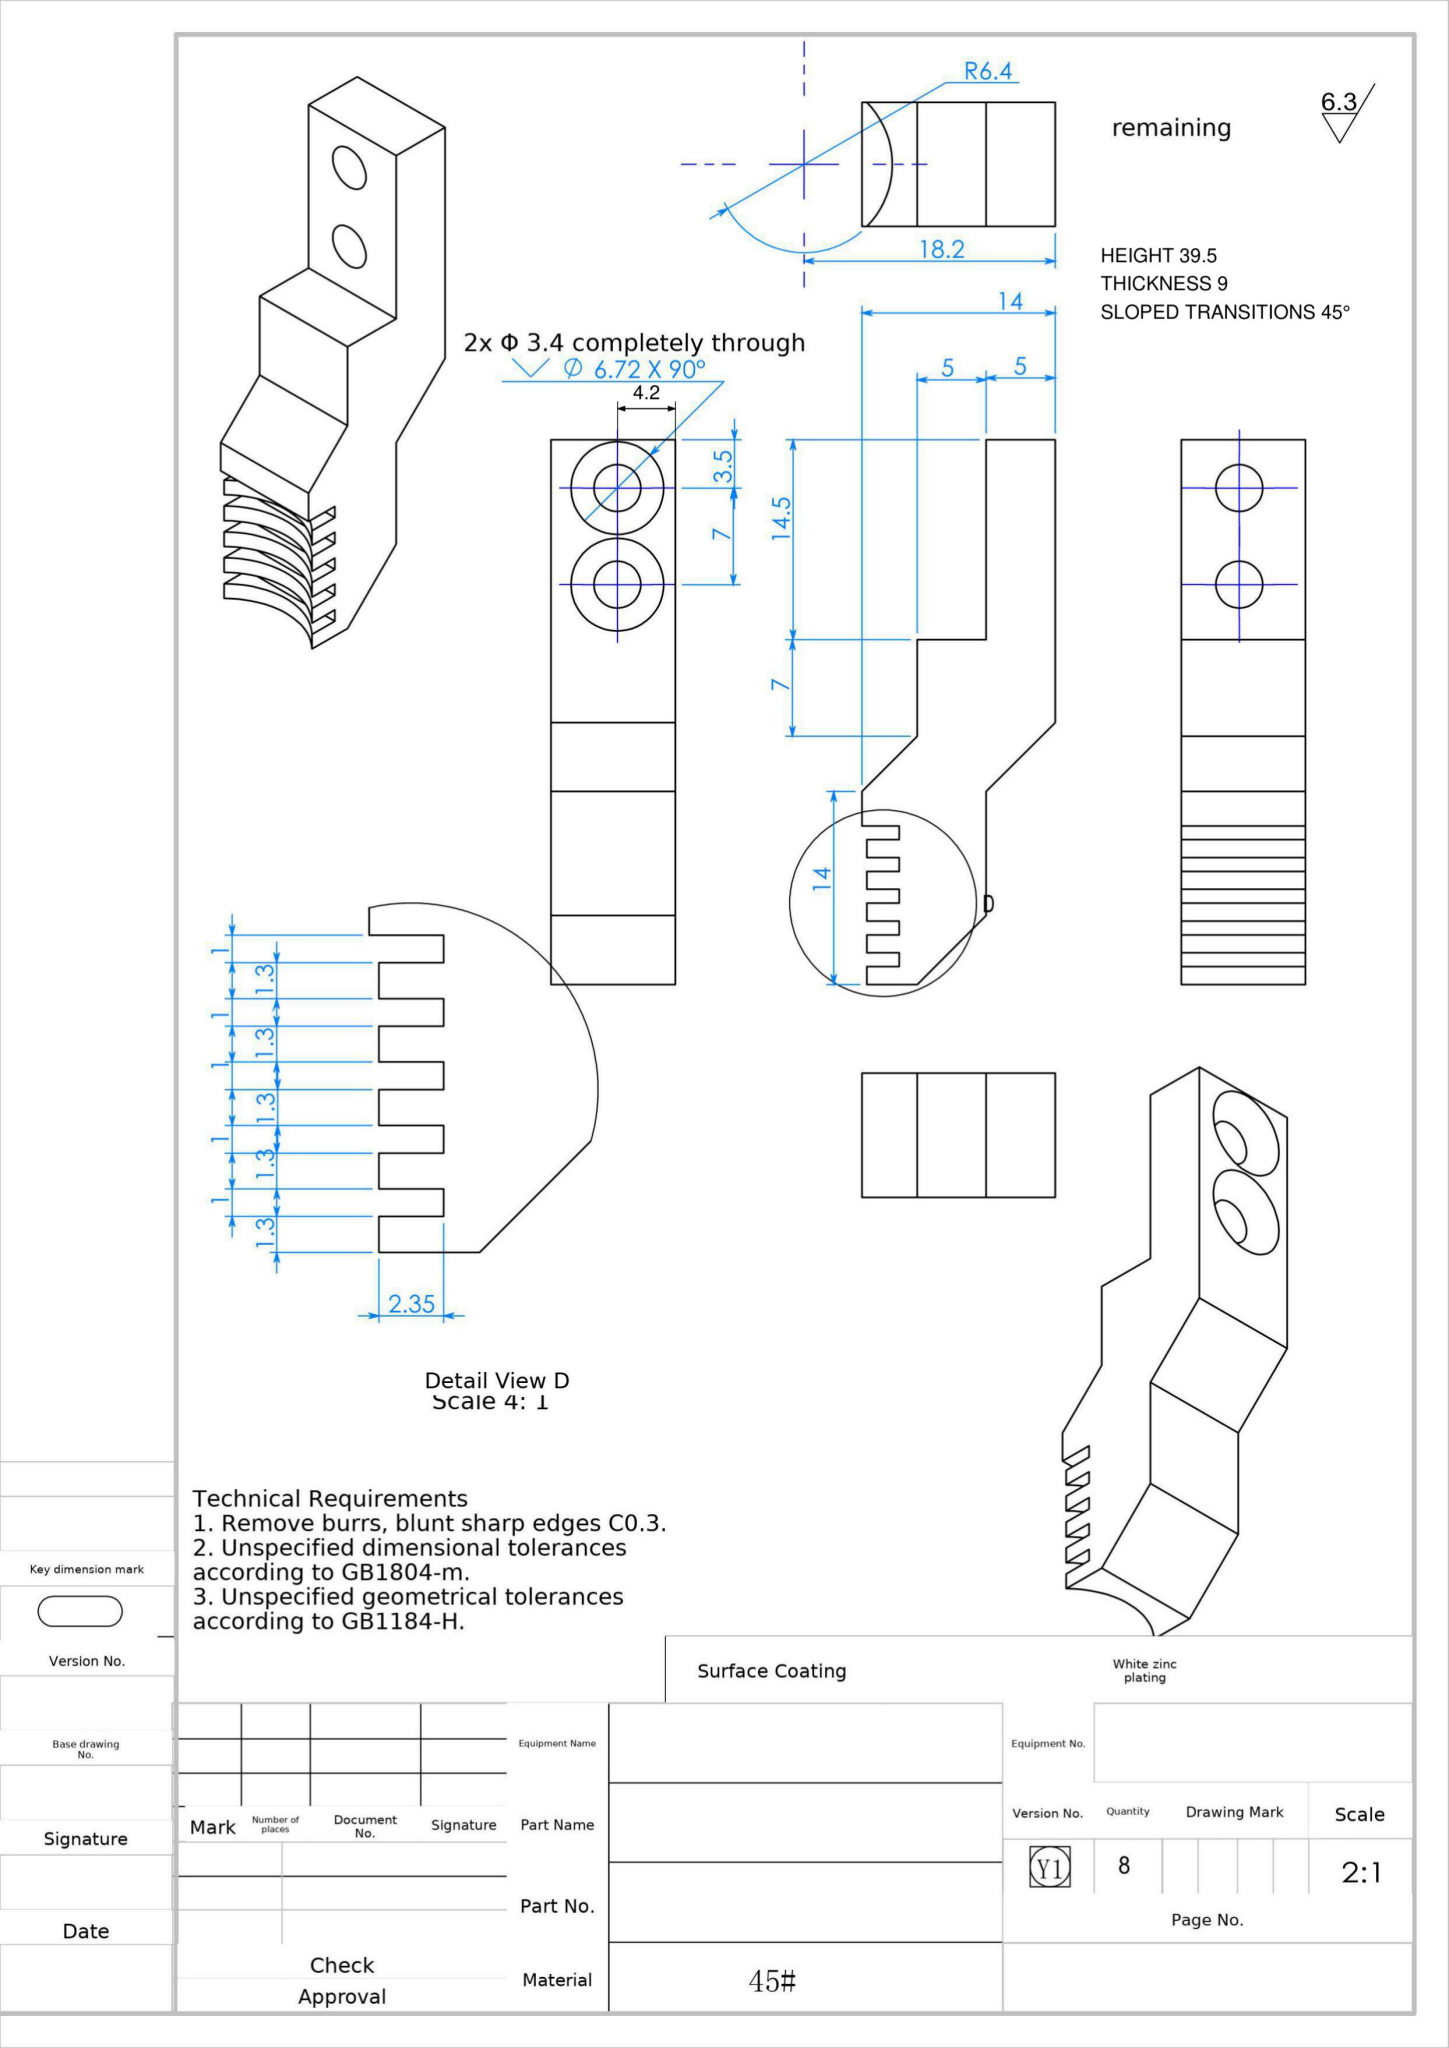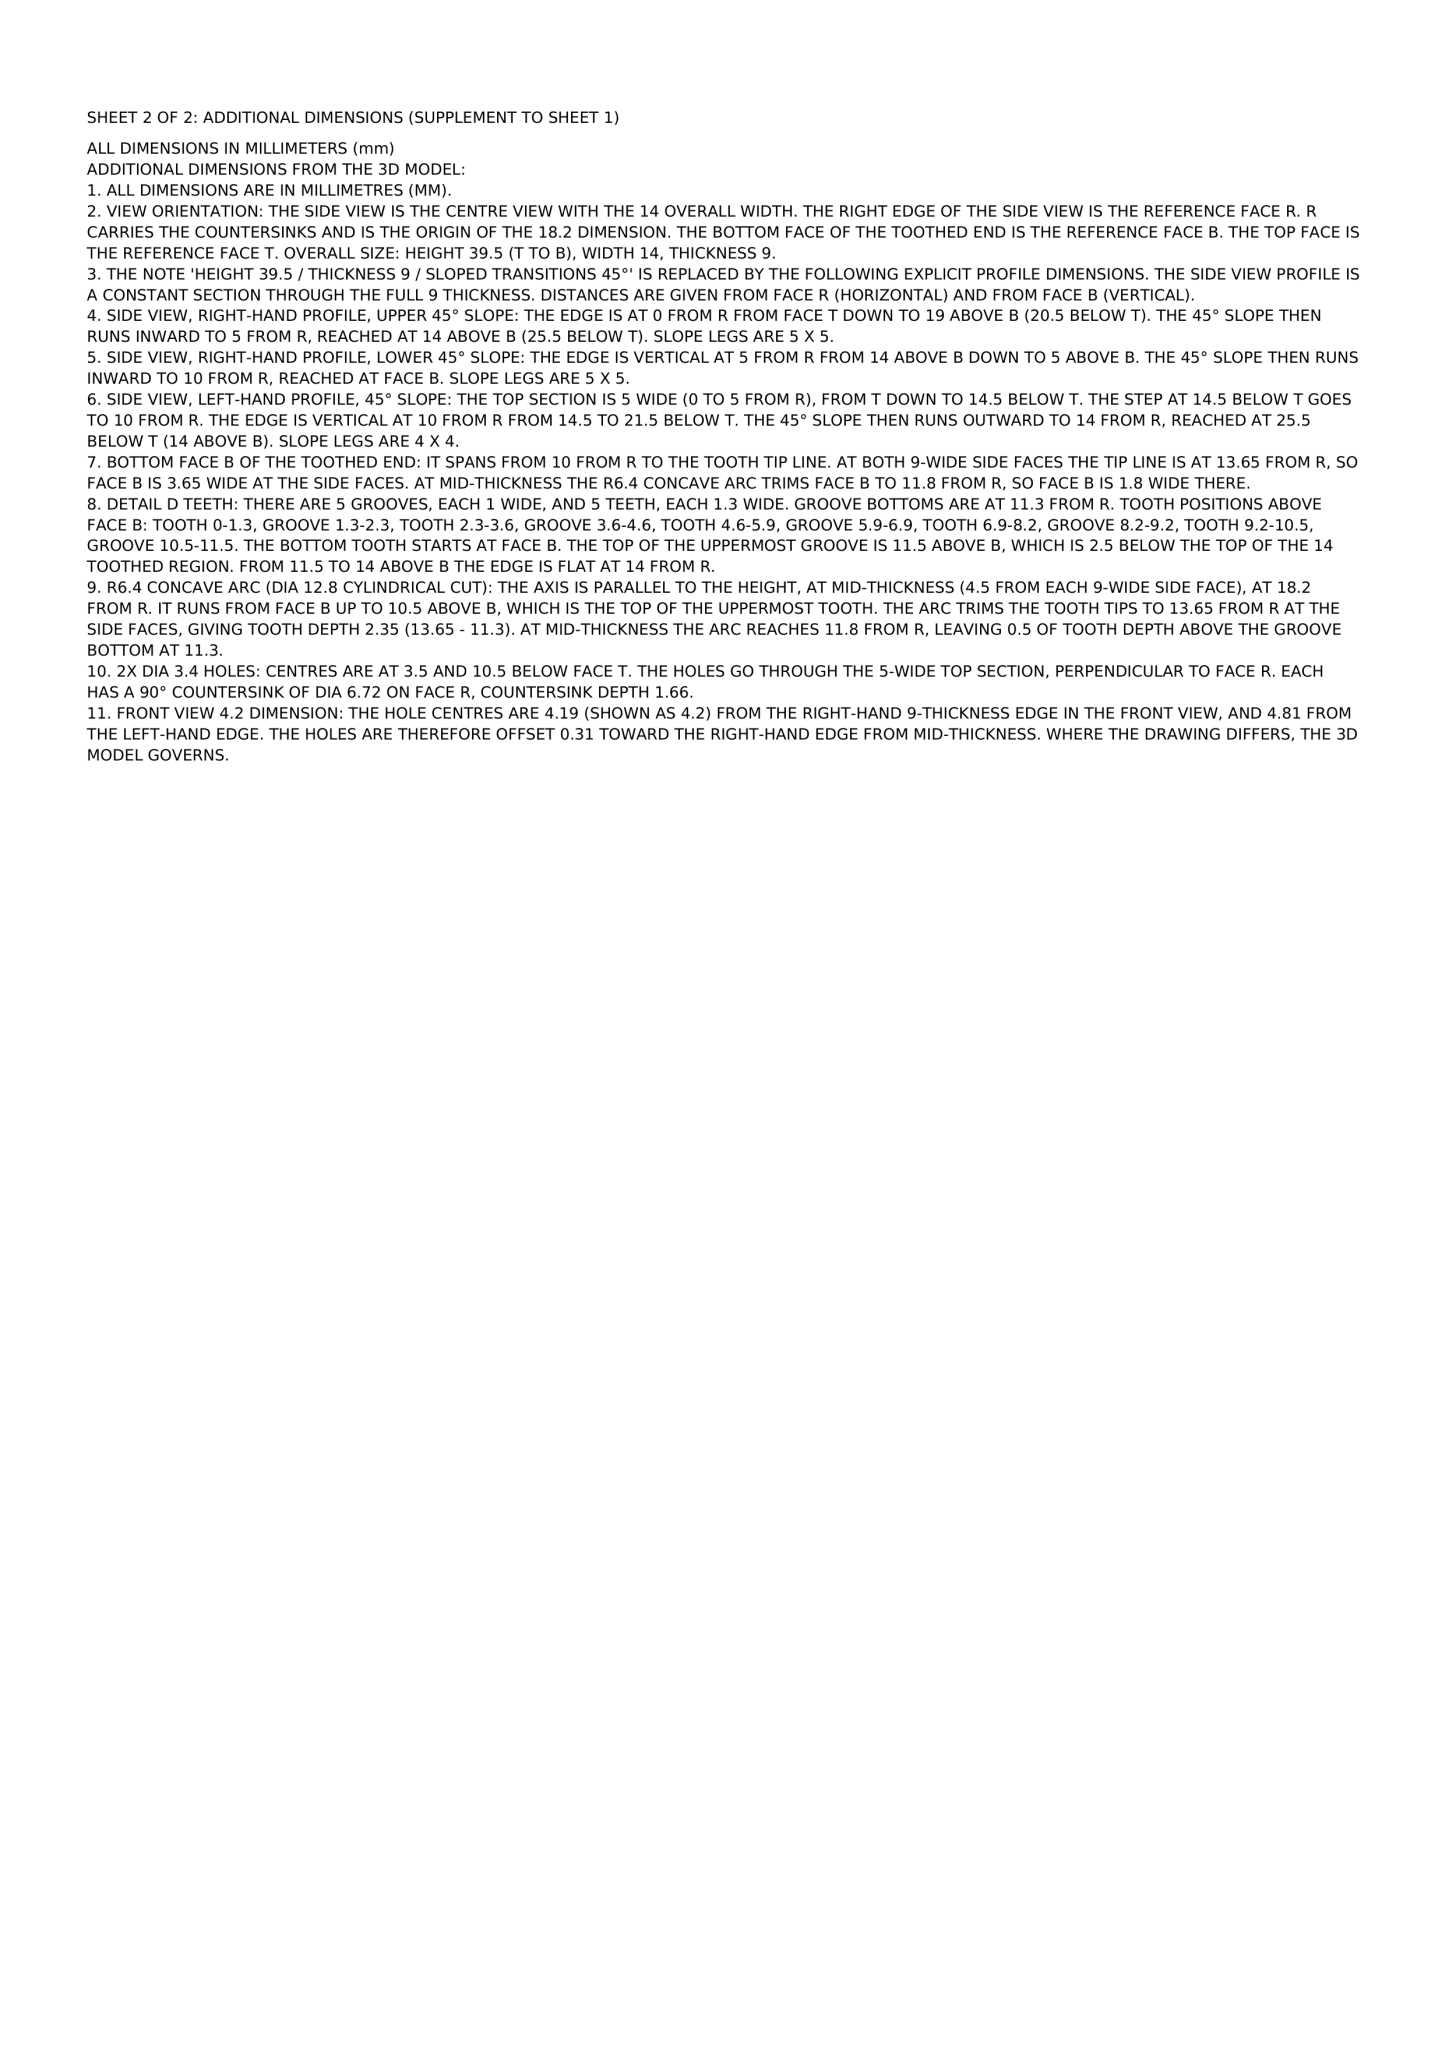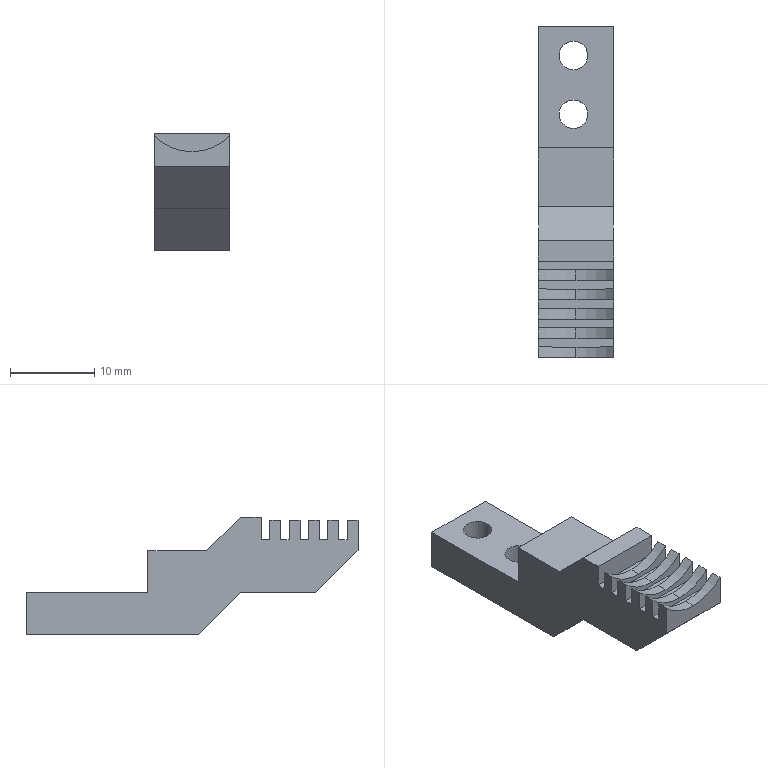Part | NX | mm | Stepped Gripper Jaw | 1 solid | 46 faces | box 9 x 39.5 x 14 mm | volume 2277 mm3 | plane 28 | cylinder 14 | cone 4 | commonest cylinder face diameters 12.8 x10 3.4 x4